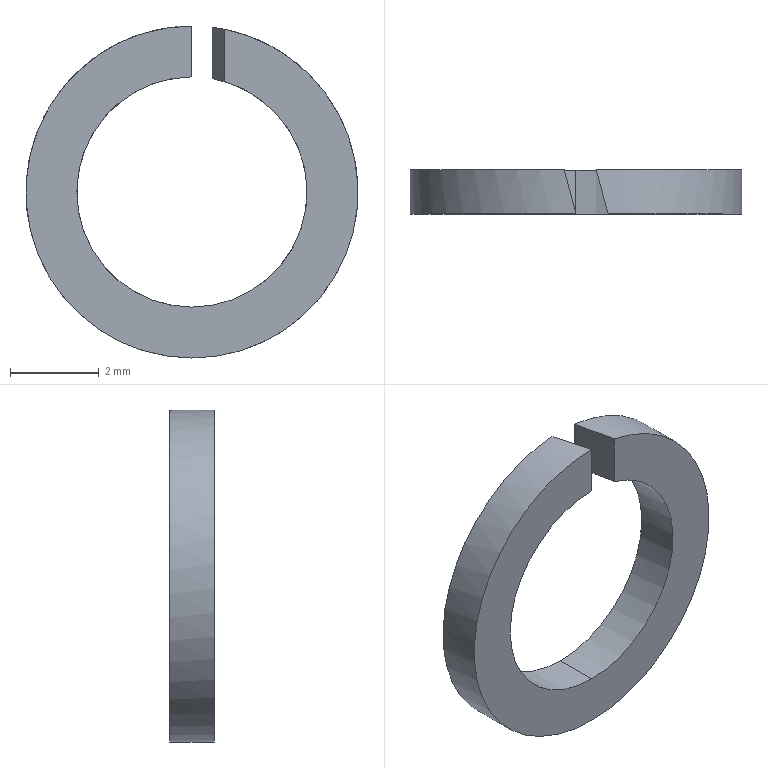Component | SolidWorks | GB 93-87-5-1 | 1 solid | 8 faces | box 7.5 x 1 x 7.5 mm | volume 22 mm3 | cylinder 4 | plane 4 | commonest cylinder face diameters 5.2 x2 7.5 x2 | material AISI 321 Annealed Stainless Steel (SS)
build123d program:
from build123d import *

# Parameters (mm, degrees)
SKETCH1_R               = 3.75
SKETCH1_R_2             = 2.6
BOSS_EXTRUDE1_DEPTH     = 1
CUT_EXTRUDE1_REACH      = 7.397
CUT_EXTRUDE1_END_RADIUS = 3.75


with BuildPart() as part:
    # Sketch1 → Boss-Extrude1 (new body)
    with BuildSketch(Plane(origin=(0, 0, 0), x_dir=(1, 0, 0), z_dir=(0, 1, 0))):
        with Locations(Location((0, 0, 0), (0, 0, 270))):
            Circle(SKETCH1_R)
        with Locations(Location((0, 0, 0), (0, 0, 270))):
            Circle(SKETCH1_R_2, mode=Mode.SUBTRACT)
    extrude(amount=BOSS_EXTRUDE1_DEPTH)

    # Cut-Extrude1: up to this cylinder (the profile starts inside it)
    cut_extrude1_end = Plane(origin=(0, 0.5, 0), z_dir=(0, -1, 0)) * Cylinder(CUT_EXTRUDE1_END_RADIUS, 23.294, mode=Mode.PRIVATE)
    # Sketch2 → Cut-Extrude1 (cut, up to the surface)
    with BuildSketch(Plane.XY, mode=Mode.PRIVATE) as cut_extrude1_sk1:
        Polygon((0, 0), (-0.2679, 1), (0.4567, 1), (0.7247, 0), align=None)
    cut_extrude1_tool1 = extrude(cut_extrude1_sk1.sketch, amount=CUT_EXTRUDE1_REACH, mode=Mode.PRIVATE) & cut_extrude1_end
    add(cut_extrude1_tool1.solids().sort_by_distance((0.2284, 0.5, 0))[0], mode=Mode.SUBTRACT)


solid = part.part

# Placed as in the assembly
solid = solid.moved(Location((-259.428, 152.796, 315.382), (0, 0, 0)))